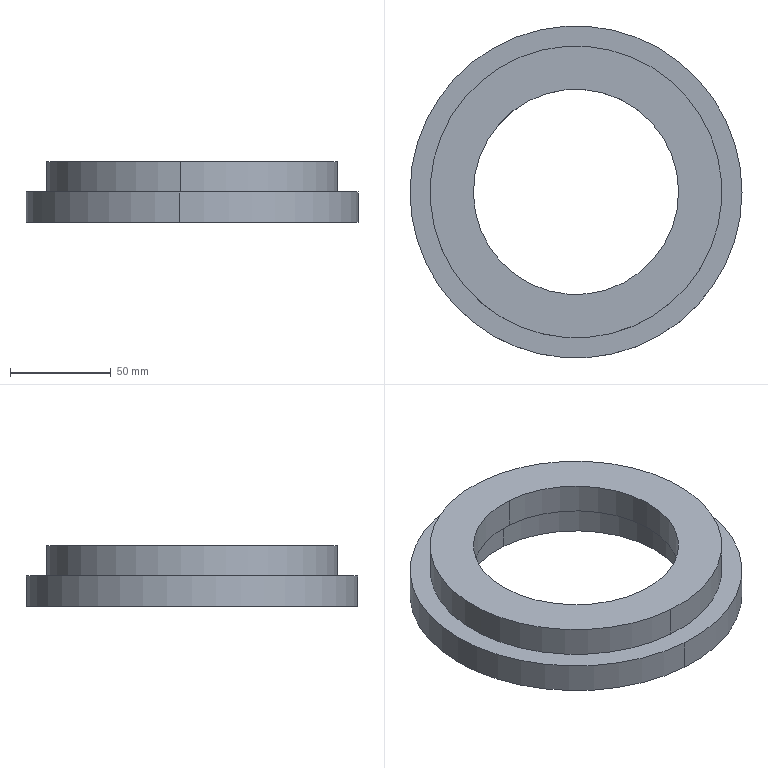Component | SolidWorks | DieRetainingRing-1 | 1 solid | 12 faces | box 165 x 165 x 30 mm | volume 303313 mm3 | cylinder 8 | plane 4 | commonest cylinder face diameters 102 x2 110 x2 145 x2 165 x2
build123d program:
from build123d import *


with BuildPart() as part:
    # Sketch1 → Revolve1 (revolve)
    with BuildSketch(Plane.XY, mode=Mode.PRIVATE) as revolve1_sk:
        Polygon((0, 0), (0, 30), (82.5, 30), (82.5, 15), (72.5, 15), (72.5, 0), align=None)
    revolve(revolve1_sk.sketch.rotate(Axis((0, 0, 0), (0, 1, 0)), 90), axis=Axis((0, 0, 0), (0, 1, 0)))

    # Sketch2 → Cut-Revolve1 (revolve, cut)
    with BuildSketch(Plane.XY, mode=Mode.PRIVATE) as cut_revolve1_sk:
        Polygon((0, 0), (0, 30), (55, 30), (55, 15), (51, 15), (51, 0), align=None)
    revolve(cut_revolve1_sk.sketch.rotate(Axis((0, 0, 0), (0, 1, 0)), 90), axis=Axis((0, 0, 0), (0, 1, 0)), mode=Mode.SUBTRACT)


solid = part.part

# Placed as in the assembly
solid = solid.moved(Location((0, 0, -216), (-90, 0, 0)))
STEP:
#1=COLOUR_RGB('',0.7922,0.8196,0.9333);
#2=FILL_AREA_STYLE_COLOUR('',#1);
#3=FILL_AREA_STYLE('',(#2));
#4=SURFACE_STYLE_FILL_AREA(#3);
#5=SURFACE_SIDE_STYLE('',(#4));
#6=SURFACE_STYLE_USAGE(.BOTH.,#5);
#7=PRESENTATION_STYLE_ASSIGNMENT((#6));
#8=CARTESIAN_POINT('',(0.1544,2.002,-9.094));
#9=VERTEX_POINT('',#8);
#10=CARTESIAN_POINT('',(-0.1544,-2.002,-9.094));
#11=VERTEX_POINT('',#10);
#12=CARTESIAN_POINT('',(-0.,0.,-9.094));
#13=DIRECTION('',(0.,0.,1.));
#14=DIRECTION('',(-0.07692,-0.997,0.));
#15=AXIS2_PLACEMENT_3D('',#12,#13,#14);
#16=CIRCLE('',#15,2.008);
#17=EDGE_CURVE('',#9,#11,#16,.T.);
#18=ORIENTED_EDGE('',*,*,#17,.F.);
#19=CARTESIAN_POINT('',(0.1544,2.002,-8.504));
#20=VERTEX_POINT('',#19);
#21=CARTESIAN_POINT('',(0.1544,2.002,-8.504));
#22=DIRECTION('',(0.,0.,1.));
#23=VECTOR('',#22,39.37);
#24=LINE('',#21,#23);
#25=EDGE_CURVE('',#9,#20,#24,.T.);
#26=ORIENTED_EDGE('',*,*,#25,.T.);
#27=CARTESIAN_POINT('',(-0.1544,-2.002,-8.504));
#28=VERTEX_POINT('',#27);
#29=CARTESIAN_POINT('',(-0.,0.,-8.504));
#30=DIRECTION('',(0.,0.,1.));
#31=DIRECTION('',(-0.07692,-0.997,0.));
#32=AXIS2_PLACEMENT_3D('',#29,#30,#31);
#33=CIRCLE('',#32,2.008);
#34=EDGE_CURVE('',#20,#28,#33,.T.);
#35=ORIENTED_EDGE('',*,*,#34,.T.);
#36=CARTESIAN_POINT('',(-0.1544,-2.002,-8.504));
#37=DIRECTION('',(0.,0.,1.));
#38=VECTOR('',#37,39.37);
#39=LINE('',#36,#38);
#40=EDGE_CURVE('',#11,#28,#39,.T.);
#41=ORIENTED_EDGE('',*,*,#40,.F.);
#42=EDGE_LOOP('',(#18,#26,#35,#41));
#43=FACE_OUTER_BOUND('',#42,.T.);
#44=CARTESIAN_POINT('',(-0.,0.,-8.504));
#45=DIRECTION('',(0.,0.,1.));
#46=DIRECTION('',(-0.07692,-0.997,0.));
#47=AXIS2_PLACEMENT_3D('',#44,#45,#46);
#48=CYLINDRICAL_SURFACE('',#47,2.008);
#49=ADVANCED_FACE('',(#43),#48,.F.);
#50=CARTESIAN_POINT('',(0.1666,2.159,-9.685));
#51=VERTEX_POINT('',#50);
#52=CARTESIAN_POINT('',(-0.1666,-2.159,-9.685));
#53=VERTEX_POINT('',#52);
#54=CARTESIAN_POINT('',(-0.,0.,-9.685));
#55=DIRECTION('',(0.,0.,1.));
#56=DIRECTION('',(-0.07692,-0.997,0.));
#57=AXIS2_PLACEMENT_3D('',#54,#55,#56);
#58=CIRCLE('',#57,2.165);
#59=EDGE_CURVE('',#51,#53,#58,.T.);
#60=ORIENTED_EDGE('',*,*,#59,.F.);
#61=CARTESIAN_POINT('',(0.1666,2.159,-9.094));
#62=VERTEX_POINT('',#61);
#63=CARTESIAN_POINT('',(0.1666,2.159,-8.504));
#64=DIRECTION('',(0.,0.,1.));
#65=VECTOR('',#64,39.37);
#66=LINE('',#63,#65);
#67=EDGE_CURVE('',#51,#62,#66,.T.);
#68=ORIENTED_EDGE('',*,*,#67,.T.);
#69=CARTESIAN_POINT('',(-0.1666,-2.159,-9.094));
#70=VERTEX_POINT('',#69);
#71=CARTESIAN_POINT('',(-0.,0.,-9.094));
#72=DIRECTION('',(0.,0.,1.));
#73=DIRECTION('',(-0.07692,-0.997,0.));
#74=AXIS2_PLACEMENT_3D('',#71,#72,#73);
#75=CIRCLE('',#74,2.165);
#76=EDGE_CURVE('',#62,#70,#75,.T.);
#77=ORIENTED_EDGE('',*,*,#76,.T.);
#78=CARTESIAN_POINT('',(-0.1666,-2.159,-8.504));
#79=DIRECTION('',(0.,0.,1.));
#80=VECTOR('',#79,39.37);
#81=LINE('',#78,#80);
#82=EDGE_CURVE('',#53,#70,#81,.T.);
#83=ORIENTED_EDGE('',*,*,#82,.F.);
#84=EDGE_LOOP('',(#60,#68,#77,#83));
#85=FACE_OUTER_BOUND('',#84,.T.);
#86=CARTESIAN_POINT('',(-0.,0.,-8.504));
#87=DIRECTION('',(0.,0.,1.));
#88=DIRECTION('',(-0.07692,-0.997,0.));
#89=AXIS2_PLACEMENT_3D('',#86,#87,#88);
#90=CYLINDRICAL_SURFACE('',#89,2.165);
#91=ADVANCED_FACE('',(#85),#90,.F.);
#92=CARTESIAN_POINT('',(-0.2196,-2.846,-9.094));
#93=VERTEX_POINT('',#92);
#94=CARTESIAN_POINT('',(0.2196,2.846,-9.094));
#95=VERTEX_POINT('',#94);
#96=CARTESIAN_POINT('',(-0.,0.,-9.094));
#97=DIRECTION('',(0.,0.,1.));
#98=DIRECTION('',(-0.07692,-0.997,0.));
#99=AXIS2_PLACEMENT_3D('',#96,#97,#98);
#100=CIRCLE('',#99,2.854);
#101=EDGE_CURVE('',#93,#95,#100,.T.);
#102=ORIENTED_EDGE('',*,*,#101,.T.);
#103=CARTESIAN_POINT('',(0.2196,2.846,-8.504));
#104=VERTEX_POINT('',#103);
#105=CARTESIAN_POINT('',(0.2196,2.846,-8.504));
#106=DIRECTION('',(0.,0.,1.));
#107=VECTOR('',#106,39.37);
#108=LINE('',#105,#107);
#109=EDGE_CURVE('',#95,#104,#108,.T.);
#110=ORIENTED_EDGE('',*,*,#109,.T.);
#111=CARTESIAN_POINT('',(-0.2196,-2.846,-8.504));
#112=VERTEX_POINT('',#111);
#113=CARTESIAN_POINT('',(-0.,0.,-8.504));
#114=DIRECTION('',(0.,0.,1.));
#115=DIRECTION('',(-0.07692,-0.997,0.));
#116=AXIS2_PLACEMENT_3D('',#113,#114,#115);
#117=CIRCLE('',#116,2.854);
#118=EDGE_CURVE('',#112,#104,#117,.T.);
#119=ORIENTED_EDGE('',*,*,#118,.F.);
#120=CARTESIAN_POINT('',(-0.2196,-2.846,-8.504));
#121=DIRECTION('',(0.,0.,1.));
#122=VECTOR('',#121,39.37);
#123=LINE('',#120,#122);
#124=EDGE_CURVE('',#93,#112,#123,.T.);
#125=ORIENTED_EDGE('',*,*,#124,.F.);
#126=EDGE_LOOP('',(#102,#110,#119,#125));
#127=FACE_OUTER_BOUND('',#126,.T.);
#128=CARTESIAN_POINT('',(-0.,0.,-8.504));
#129=DIRECTION('',(0.,0.,1.));
#130=DIRECTION('',(-0.07692,-0.997,0.));
#131=AXIS2_PLACEMENT_3D('',#128,#129,#130);
#132=CYLINDRICAL_SURFACE('',#131,2.854);
#133=ADVANCED_FACE('',(#127),#132,.T.);
#134=CARTESIAN_POINT('',(-0.2498,-3.238,-9.685));
#135=VERTEX_POINT('',#134);
#136=CARTESIAN_POINT('',(0.2498,3.238,-9.685));
#137=VERTEX_POINT('',#136);
#138=CARTESIAN_POINT('',(-0.,0.,-9.685));
#139=DIRECTION('',(0.,0.,1.));
#140=DIRECTION('',(-0.07692,-0.997,0.));
#141=AXIS2_PLACEMENT_3D('',#138,#139,#140);
#142=CIRCLE('',#141,3.248);
#143=EDGE_CURVE('',#135,#137,#142,.T.);
#144=ORIENTED_EDGE('',*,*,#143,.T.);
#145=CARTESIAN_POINT('',(0.2498,3.238,-9.094));
#146=VERTEX_POINT('',#145);
#147=CARTESIAN_POINT('',(0.2498,3.238,-8.504));
#148=DIRECTION('',(0.,0.,1.));
#149=VECTOR('',#148,39.37);
#150=LINE('',#147,#149);
#151=EDGE_CURVE('',#137,#146,#150,.T.);
#152=ORIENTED_EDGE('',*,*,#151,.T.);
#153=CARTESIAN_POINT('',(-0.2498,-3.238,-9.094));
#154=VERTEX_POINT('',#153);
#155=CARTESIAN_POINT('',(-0.,0.,-9.094));
#156=DIRECTION('',(0.,0.,1.));
#157=DIRECTION('',(-0.07692,-0.997,0.));
#158=AXIS2_PLACEMENT_3D('',#155,#156,#157);
#159=CIRCLE('',#158,3.248);
#160=EDGE_CURVE('',#154,#146,#159,.T.);
#161=ORIENTED_EDGE('',*,*,#160,.F.);
#162=CARTESIAN_POINT('',(-0.2498,-3.238,-8.504));
#163=DIRECTION('',(0.,0.,1.));
#164=VECTOR('',#163,39.37);
#165=LINE('',#162,#164);
#166=EDGE_CURVE('',#135,#154,#165,.T.);
#167=ORIENTED_EDGE('',*,*,#166,.F.);
#168=EDGE_LOOP('',(#144,#152,#161,#167));
#169=FACE_OUTER_BOUND('',#168,.T.);
#170=CARTESIAN_POINT('',(-0.,0.,-8.504));
#171=DIRECTION('',(0.,0.,1.));
#172=DIRECTION('',(-0.07692,-0.997,0.));
#173=AXIS2_PLACEMENT_3D('',#170,#171,#172);
#174=CYLINDRICAL_SURFACE('',#173,3.248);
#175=ADVANCED_FACE('',(#169),#174,.T.);
#176=CARTESIAN_POINT('',(-0.,0.,-8.504));
#177=DIRECTION('',(0.,0.,1.));
#178=DIRECTION('',(-0.07692,-0.997,0.));
#179=AXIS2_PLACEMENT_3D('',#176,#177,#178);
#180=CIRCLE('',#179,2.008);
#181=EDGE_CURVE('',#28,#20,#180,.T.);
#182=ORIENTED_EDGE('',*,*,#181,.F.);
#183=ORIENTED_EDGE('',*,*,#34,.F.);
#184=EDGE_LOOP('',(#182,#183));
#185=FACE_BOUND('',#184,.T.);
#186=ORIENTED_EDGE('',*,*,#118,.T.);
#187=CARTESIAN_POINT('',(-0.,0.,-8.504));
#188=DIRECTION('',(0.,0.,1.));
#189=DIRECTION('',(-0.07692,-0.997,0.));
#190=AXIS2_PLACEMENT_3D('',#187,#188,#189);
#191=CIRCLE('',#190,2.854);
#192=EDGE_CURVE('',#104,#112,#191,.T.);
#193=ORIENTED_EDGE('',*,*,#192,.T.);
#194=EDGE_LOOP('',(#186,#193));
#195=FACE_OUTER_BOUND('',#194,.T.);
#196=CARTESIAN_POINT('',(2.846,-0.2196,-8.504));
#197=DIRECTION('',(0.,0.,1.));
#198=DIRECTION('',(-0.07692,-0.997,0.));
#199=AXIS2_PLACEMENT_3D('',#196,#197,#198);
#200=PLANE('',#199);
#201=ADVANCED_FACE('',(#185,#195),#200,.T.);
#202=CARTESIAN_POINT('',(-0.,0.,-9.685));
#203=DIRECTION('',(0.,0.,1.));
#204=DIRECTION('',(-0.07692,-0.997,0.));
#205=AXIS2_PLACEMENT_3D('',#202,#203,#204);
#206=CIRCLE('',#205,2.165);
#207=EDGE_CURVE('',#53,#51,#206,.T.);
#208=ORIENTED_EDGE('',*,*,#207,.T.);
#209=ORIENTED_EDGE('',*,*,#59,.T.);
#210=EDGE_LOOP('',(#208,#209));
#211=FACE_BOUND('',#210,.T.);
#212=ORIENTED_EDGE('',*,*,#143,.F.);
#213=CARTESIAN_POINT('',(-0.,0.,-9.685));
#214=DIRECTION('',(0.,0.,1.));
#215=DIRECTION('',(-0.07692,-0.997,0.));
#216=AXIS2_PLACEMENT_3D('',#213,#214,#215);
#217=CIRCLE('',#216,3.248);
#218=EDGE_CURVE('',#137,#135,#217,.T.);
#219=ORIENTED_EDGE('',*,*,#218,.F.);
#220=EDGE_LOOP('',(#212,#219));
#221=FACE_OUTER_BOUND('',#220,.T.);
#222=CARTESIAN_POINT('',(-0.,0.,-9.685));
#223=DIRECTION('',(0.,0.,-1.));
#224=DIRECTION('',(0.07692,0.997,0.));
#225=AXIS2_PLACEMENT_3D('',#222,#223,#224);
#226=PLANE('',#225);
#227=ADVANCED_FACE('',(#211,#221),#226,.T.);
#228=ORIENTED_EDGE('',*,*,#151,.F.);
#229=ORIENTED_EDGE('',*,*,#218,.T.);
#230=ORIENTED_EDGE('',*,*,#166,.T.);
#231=CARTESIAN_POINT('',(-0.,0.,-9.094));
#232=DIRECTION('',(0.,0.,1.));
#233=DIRECTION('',(-0.07692,-0.997,0.));
#234=AXIS2_PLACEMENT_3D('',#231,#232,#233);
#235=CIRCLE('',#234,3.248);
#236=EDGE_CURVE('',#146,#154,#235,.T.);
#237=ORIENTED_EDGE('',*,*,#236,.F.);
#238=EDGE_LOOP('',(#228,#229,#230,#237));
#239=FACE_OUTER_BOUND('',#238,.T.);
#240=CARTESIAN_POINT('',(-0.,0.,-8.504));
#241=DIRECTION('',(0.,0.,1.));
#242=DIRECTION('',(-0.07692,-0.997,0.));
#243=AXIS2_PLACEMENT_3D('',#240,#241,#242);
#244=CYLINDRICAL_SURFACE('',#243,3.248);
#245=ADVANCED_FACE('',(#239),#244,.T.);
#246=ORIENTED_EDGE('',*,*,#160,.T.);
#247=ORIENTED_EDGE('',*,*,#236,.T.);
#248=EDGE_LOOP('',(#246,#247));
#249=FACE_OUTER_BOUND('',#248,.T.);
#250=ORIENTED_EDGE('',*,*,#101,.F.);
#251=CARTESIAN_POINT('',(-0.,0.,-9.094));
#252=DIRECTION('',(0.,0.,1.));
#253=DIRECTION('',(-0.07692,-0.997,0.));
#254=AXIS2_PLACEMENT_3D('',#251,#252,#253);
#255=CIRCLE('',#254,2.854);
#256=EDGE_CURVE('',#95,#93,#255,.T.);
#257=ORIENTED_EDGE('',*,*,#256,.F.);
#258=EDGE_LOOP('',(#250,#257));
#259=FACE_BOUND('',#258,.T.);
#260=CARTESIAN_POINT('',(3.238,-0.2498,-9.094));
#261=DIRECTION('',(0.,0.,1.));
#262=DIRECTION('',(-0.07692,-0.997,0.));
#263=AXIS2_PLACEMENT_3D('',#260,#261,#262);
#264=PLANE('',#263);
#265=ADVANCED_FACE('',(#249,#259),#264,.T.);
#266=ORIENTED_EDGE('',*,*,#109,.F.);
#267=ORIENTED_EDGE('',*,*,#256,.T.);
#268=ORIENTED_EDGE('',*,*,#124,.T.);
#269=ORIENTED_EDGE('',*,*,#192,.F.);
#270=EDGE_LOOP('',(#266,#267,#268,#269));
#271=FACE_OUTER_BOUND('',#270,.T.);
#272=CARTESIAN_POINT('',(-0.,0.,-8.504));
#273=DIRECTION('',(0.,0.,1.));
#274=DIRECTION('',(-0.07692,-0.997,0.));
#275=AXIS2_PLACEMENT_3D('',#272,#273,#274);
#276=CYLINDRICAL_SURFACE('',#275,2.854);
#277=ADVANCED_FACE('',(#271),#276,.T.);
#278=ORIENTED_EDGE('',*,*,#67,.F.);
#279=ORIENTED_EDGE('',*,*,#207,.F.);
#280=ORIENTED_EDGE('',*,*,#82,.T.);
#281=CARTESIAN_POINT('',(-0.,0.,-9.094));
#282=DIRECTION('',(0.,0.,1.));
#283=DIRECTION('',(-0.07692,-0.997,0.));
#284=AXIS2_PLACEMENT_3D('',#281,#282,#283);
#285=CIRCLE('',#284,2.165);
#286=EDGE_CURVE('',#70,#62,#285,.T.);
#287=ORIENTED_EDGE('',*,*,#286,.T.);
#288=EDGE_LOOP('',(#278,#279,#280,#287));
#289=FACE_OUTER_BOUND('',#288,.T.);
#290=CARTESIAN_POINT('',(-0.,0.,-8.504));
#291=DIRECTION('',(0.,0.,1.));
#292=DIRECTION('',(-0.07692,-0.997,0.));
#293=AXIS2_PLACEMENT_3D('',#290,#291,#292);
#294=CYLINDRICAL_SURFACE('',#293,2.165);
#295=ADVANCED_FACE('',(#289),#294,.F.);
#296=ORIENTED_EDGE('',*,*,#286,.F.);
#297=ORIENTED_EDGE('',*,*,#76,.F.);
#298=EDGE_LOOP('',(#296,#297));
#299=FACE_OUTER_BOUND('',#298,.T.);
#300=CARTESIAN_POINT('',(-0.,0.,-9.094));
#301=DIRECTION('',(0.,0.,1.));
#302=DIRECTION('',(-0.07692,-0.997,0.));
#303=AXIS2_PLACEMENT_3D('',#300,#301,#302);
#304=CIRCLE('',#303,2.008);
#305=EDGE_CURVE('',#11,#9,#304,.T.);
#306=ORIENTED_EDGE('',*,*,#305,.T.);
#307=ORIENTED_EDGE('',*,*,#17,.T.);
#308=EDGE_LOOP('',(#306,#307));
#309=FACE_BOUND('',#308,.T.);
#310=CARTESIAN_POINT('',(2.159,-0.1666,-9.094));
#311=DIRECTION('',(0.,0.,1.));
#312=DIRECTION('',(-0.07692,-0.997,0.));
#313=AXIS2_PLACEMENT_3D('',#310,#311,#312);
#314=PLANE('',#313);
#315=ADVANCED_FACE('',(#299,#309),#314,.F.);
#316=ORIENTED_EDGE('',*,*,#25,.F.);
#317=ORIENTED_EDGE('',*,*,#305,.F.);
#318=ORIENTED_EDGE('',*,*,#40,.T.);
#319=ORIENTED_EDGE('',*,*,#181,.T.);
#320=EDGE_LOOP('',(#316,#317,#318,#319));
#321=FACE_OUTER_BOUND('',#320,.T.);
#322=CARTESIAN_POINT('',(-0.,0.,-8.504));
#323=DIRECTION('',(0.,0.,1.));
#324=DIRECTION('',(-0.07692,-0.997,0.));
#325=AXIS2_PLACEMENT_3D('',#322,#323,#324);
#326=CYLINDRICAL_SURFACE('',#325,2.008);
#327=ADVANCED_FACE('',(#321),#326,.F.);
#328=CLOSED_SHELL('',(#49,#91,#133,#175,#201,#227,#245,#265,#277,#295,#315,#327));
#329=MANIFOLD_SOLID_BREP('',#328);
#330=STYLED_ITEM('',(#7),#329);
#331=(LENGTH_UNIT()NAMED_UNIT(*)SI_UNIT($,.METRE.));
#332=LENGTH_MEASURE_WITH_UNIT(LENGTH_MEASURE(0.0254),#331);
#333=DIMENSIONAL_EXPONENTS(1.,0.,0.,0.,0.,0.,0.);
#334=(CONVERSION_BASED_UNIT('',#332)LENGTH_UNIT()NAMED_UNIT(#333));
#335=UNCERTAINTY_MEASURE_WITH_UNIT(LENGTH_MEASURE(0.00001),#334,'','');
#336=(NAMED_UNIT(*)PLANE_ANGLE_UNIT()SI_UNIT($,.RADIAN.));
#337=(NAMED_UNIT(*)SI_UNIT($,.STERADIAN.)SOLID_ANGLE_UNIT());
#338=(GEOMETRIC_REPRESENTATION_CONTEXT(3)GLOBAL_UNCERTAINTY_ASSIGNED_CONTEXT((#335))GLOBAL_UNIT_ASSIGNED_CONTEXT((#334,#336,#337))REPRESENTATION_CONTEXT('',''));
#339=MECHANICAL_DESIGN_GEOMETRIC_PRESENTATION_REPRESENTATION('',(#330),#338);
#340=PRESENTATION_LAYER_ASSIGNMENT('','',(#330));
#341=CARTESIAN_POINT('',(0.,0.,0.));
#342=DIRECTION('',(0.,0.,1.));
#343=DIRECTION('',(1.,0.,0.));
#344=AXIS2_PLACEMENT_3D('',#341,#342,#343);
#345=(LENGTH_UNIT()NAMED_UNIT(*)SI_UNIT($,.METRE.));
#346=LENGTH_MEASURE_WITH_UNIT(LENGTH_MEASURE(0.0254),#345);
#347=DIMENSIONAL_EXPONENTS(1.,0.,0.,0.,0.,0.,0.);
#348=(CONVERSION_BASED_UNIT('',#346)LENGTH_UNIT()NAMED_UNIT(#347));
#349=UNCERTAINTY_MEASURE_WITH_UNIT(LENGTH_MEASURE(0.00001),#348,'','');
#350=(NAMED_UNIT(*)PLANE_ANGLE_UNIT()SI_UNIT($,.RADIAN.));
#351=(NAMED_UNIT(*)SI_UNIT($,.STERADIAN.)SOLID_ANGLE_UNIT());
#352=(GEOMETRIC_REPRESENTATION_CONTEXT(3)GLOBAL_UNCERTAINTY_ASSIGNED_CONTEXT((#349))GLOBAL_UNIT_ASSIGNED_CONTEXT((#348,#350,#351))REPRESENTATION_CONTEXT('',''));
#353=ADVANCED_BREP_SHAPE_REPRESENTATION('',(#329,#344),#352);